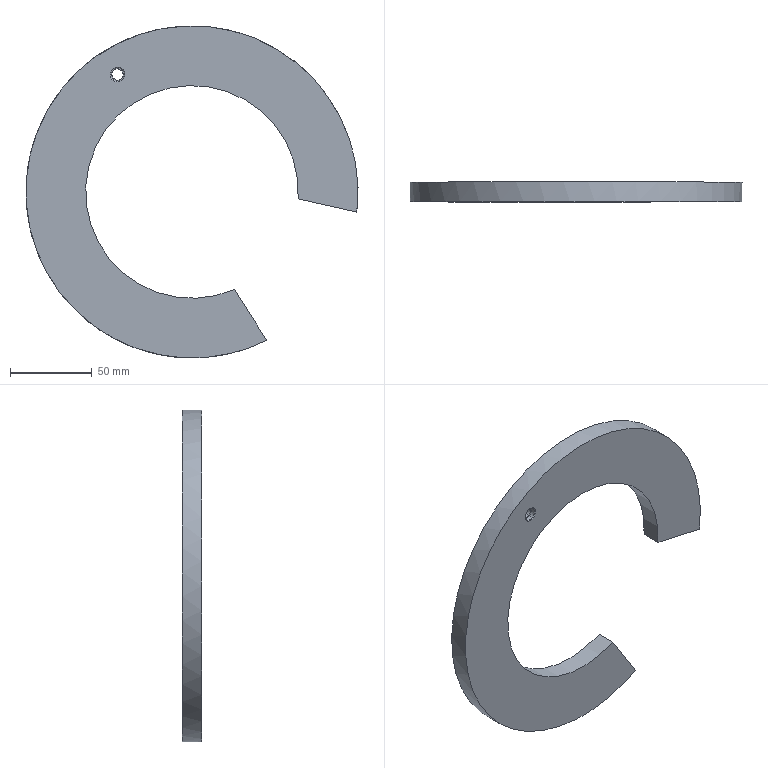Component | SolidWorks | Turntable-1 | 1 solid | 13 faces | box 203 x 12 x 203 mm | volume 191203 mm3 | cylinder 6 | plane 5 | cone 2 | commonest cylinder face diameters 8 x2 6.8 x2 130 x1 203 x1
STEP:
#1=CARTESIAN_POINT('',(1.076,-1.949,9.179));
#2=VERTEX_POINT('',#1);
#3=CARTESIAN_POINT('',(1.245,-1.949,8.913));
#4=VERTEX_POINT('',#3);
#5=CARTESIAN_POINT('',(1.16,-1.949,9.046));
#6=DIRECTION('',(0.,-1.,0.));
#7=DIRECTION('',(0.5356,0.,-0.8445));
#8=AXIS2_PLACEMENT_3D('',#5,#6,#7);
#9=CIRCLE('',#8,0.1575);
#10=EDGE_CURVE('',#2,#4,#9,.T.);
#11=ORIENTED_EDGE('',*,*,#10,.F.);
#12=CARTESIAN_POINT('',(1.076,-2.05,9.179));
#13=VERTEX_POINT('',#12);
#14=CARTESIAN_POINT('',(1.076,-1.949,9.179));
#15=DIRECTION('',(0.,-1.,0.));
#16=VECTOR('',#15,39.37);
#17=LINE('',#14,#16);
#18=EDGE_CURVE('',#2,#13,#17,.T.);
#19=ORIENTED_EDGE('',*,*,#18,.T.);
#20=CARTESIAN_POINT('',(1.245,-2.05,8.913));
#21=VERTEX_POINT('',#20);
#22=CARTESIAN_POINT('',(1.16,-2.05,9.046));
#23=DIRECTION('',(0.,1.,0.));
#24=DIRECTION('',(0.5356,0.,-0.8445));
#25=AXIS2_PLACEMENT_3D('',#22,#23,#24);
#26=CIRCLE('',#25,0.1575);
#27=EDGE_CURVE('',#21,#13,#26,.T.);
#28=ORIENTED_EDGE('',*,*,#27,.F.);
#29=CARTESIAN_POINT('',(1.245,-1.949,8.913));
#30=DIRECTION('',(0.,-1.,0.));
#31=VECTOR('',#30,39.37);
#32=LINE('',#29,#31);
#33=EDGE_CURVE('',#4,#21,#32,.T.);
#34=ORIENTED_EDGE('',*,*,#33,.F.);
#35=EDGE_LOOP('',(#11,#19,#28,#34));
#36=FACE_OUTER_BOUND('',#35,.T.);
#37=CARTESIAN_POINT('',(1.16,-1.949,9.046));
#38=DIRECTION('',(0.,-1.,0.));
#39=DIRECTION('',(0.5356,0.,-0.8445));
#40=AXIS2_PLACEMENT_3D('',#37,#38,#39);
#41=CYLINDRICAL_SURFACE('',#40,0.1575);
#42=ADVANCED_FACE('',(#36),#41,.F.);
#43=ORIENTED_EDGE('',*,*,#27,.T.);
#44=CARTESIAN_POINT('',(1.065,-2.067,9.197));
#45=VERTEX_POINT('',#44);
#46=CARTESIAN_POINT('',(1.065,-2.067,9.197));
#47=DIRECTION('',(-0.4103,-0.6428,0.6469));
#48=VECTOR('',#47,39.37);
#49=LINE('',#46,#48);
#50=EDGE_CURVE('',#13,#45,#49,.T.);
#51=ORIENTED_EDGE('',*,*,#50,.T.);
#52=CARTESIAN_POINT('',(1.256,-2.067,8.896));
#53=VERTEX_POINT('',#52);
#54=CARTESIAN_POINT('',(1.16,-2.067,9.046));
#55=DIRECTION('',(0.,-1.,0.));
#56=DIRECTION('',(0.5356,0.,-0.8445));
#57=AXIS2_PLACEMENT_3D('',#54,#55,#56);
#58=CIRCLE('',#57,0.1781);
#59=EDGE_CURVE('',#45,#53,#58,.T.);
#60=ORIENTED_EDGE('',*,*,#59,.T.);
#61=CARTESIAN_POINT('',(1.256,-2.067,8.896));
#62=DIRECTION('',(0.4103,-0.6428,-0.6469));
#63=VECTOR('',#62,39.37);
#64=LINE('',#61,#63);
#65=EDGE_CURVE('',#21,#53,#64,.T.);
#66=ORIENTED_EDGE('',*,*,#65,.F.);
#67=EDGE_LOOP('',(#43,#51,#60,#66));
#68=FACE_OUTER_BOUND('',#67,.T.);
#69=CARTESIAN_POINT('',(1.16,-2.067,9.046));
#70=DIRECTION('',(0.,-1.,0.));
#71=DIRECTION('',(0.5356,0.,-0.8445));
#72=AXIS2_PLACEMENT_3D('',#69,#70,#71);
#73=CONICAL_SURFACE('',#72,0.1781,0.8727);
#74=ADVANCED_FACE('',(#68),#73,.F.);
#75=CARTESIAN_POINT('',(1.089,-1.594,9.16));
#76=VERTEX_POINT('',#75);
#77=CARTESIAN_POINT('',(1.232,-1.594,8.933));
#78=VERTEX_POINT('',#77);
#79=CARTESIAN_POINT('',(1.16,-1.594,9.046));
#80=DIRECTION('',(0.,-1.,0.));
#81=DIRECTION('',(0.5356,0.,-0.8445));
#82=AXIS2_PLACEMENT_3D('',#79,#80,#81);
#83=CIRCLE('',#82,0.1339);
#84=EDGE_CURVE('',#76,#78,#83,.T.);
#85=ORIENTED_EDGE('',*,*,#84,.F.);
#86=CARTESIAN_POINT('',(1.089,-1.949,9.16));
#87=VERTEX_POINT('',#86);
#88=CARTESIAN_POINT('',(1.089,-2.067,9.16));
#89=DIRECTION('',(0.,-1.,0.));
#90=VECTOR('',#89,39.37);
#91=LINE('',#88,#90);
#92=EDGE_CURVE('',#76,#87,#91,.T.);
#93=ORIENTED_EDGE('',*,*,#92,.T.);
#94=CARTESIAN_POINT('',(1.232,-1.949,8.933));
#95=VERTEX_POINT('',#94);
#96=CARTESIAN_POINT('',(1.16,-1.949,9.046));
#97=DIRECTION('',(0.,1.,0.));
#98=DIRECTION('',(0.5356,0.,-0.8445));
#99=AXIS2_PLACEMENT_3D('',#96,#97,#98);
#100=CIRCLE('',#99,0.1339);
#101=EDGE_CURVE('',#95,#87,#100,.T.);
#102=ORIENTED_EDGE('',*,*,#101,.F.);
#103=CARTESIAN_POINT('',(1.232,-2.067,8.933));
#104=DIRECTION('',(0.,-1.,0.));
#105=VECTOR('',#104,39.37);
#106=LINE('',#103,#105);
#107=EDGE_CURVE('',#78,#95,#106,.T.);
#108=ORIENTED_EDGE('',*,*,#107,.F.);
#109=EDGE_LOOP('',(#85,#93,#102,#108));
#110=FACE_OUTER_BOUND('',#109,.T.);
#111=CARTESIAN_POINT('',(1.16,-2.067,9.046));
#112=DIRECTION('',(0.,-1.,0.));
#113=DIRECTION('',(0.5356,0.,-0.8445));
#114=AXIS2_PLACEMENT_3D('',#111,#112,#113);
#115=CYLINDRICAL_SURFACE('',#114,0.1339);
#116=ADVANCED_FACE('',(#110),#115,.F.);
#117=ORIENTED_EDGE('',*,*,#92,.F.);
#118=CARTESIAN_POINT('',(1.16,-1.594,9.046));
#119=DIRECTION('',(0.,-1.,0.));
#120=DIRECTION('',(0.5356,0.,-0.8445));
#121=AXIS2_PLACEMENT_3D('',#118,#119,#120);
#122=CIRCLE('',#121,0.1339);
#123=EDGE_CURVE('',#78,#76,#122,.T.);
#124=ORIENTED_EDGE('',*,*,#123,.F.);
#125=ORIENTED_EDGE('',*,*,#107,.T.);
#126=CARTESIAN_POINT('',(1.16,-1.949,9.046));
#127=DIRECTION('',(0.,1.,0.));
#128=DIRECTION('',(0.5356,0.,-0.8445));
#129=AXIS2_PLACEMENT_3D('',#126,#127,#128);
#130=CIRCLE('',#129,0.1339);
#131=EDGE_CURVE('',#87,#95,#130,.T.);
#132=ORIENTED_EDGE('',*,*,#131,.F.);
#133=EDGE_LOOP('',(#117,#124,#125,#132));
#134=FACE_OUTER_BOUND('',#133,.T.);
#135=CARTESIAN_POINT('',(1.16,-2.067,9.046));
#136=DIRECTION('',(0.,-1.,0.));
#137=DIRECTION('',(0.5356,0.,-0.8445));
#138=AXIS2_PLACEMENT_3D('',#135,#136,#137);
#139=CYLINDRICAL_SURFACE('',#138,0.1339);
#140=ADVANCED_FACE('',(#134),#139,.F.);
#141=CARTESIAN_POINT('',(1.16,-2.067,9.046));
#142=DIRECTION('',(0.,-1.,0.));
#143=DIRECTION('',(0.5356,0.,-0.8445));
#144=AXIS2_PLACEMENT_3D('',#141,#142,#143);
#145=CIRCLE('',#144,0.1781);
#146=EDGE_CURVE('',#53,#45,#145,.T.);
#147=ORIENTED_EDGE('',*,*,#146,.F.);
#148=ORIENTED_EDGE('',*,*,#59,.F.);
#149=EDGE_LOOP('',(#147,#148));
#150=FACE_BOUND('',#149,.T.);
#151=CARTESIAN_POINT('',(6.919,-2.067,5.736));
#152=VERTEX_POINT('',#151);
#153=CARTESIAN_POINT('',(5.506,-2.067,6.052));
#154=VERTEX_POINT('',#153);
#155=CARTESIAN_POINT('',(5.506,-2.067,6.052));
#156=DIRECTION('',(-0.9759,0.,0.2184));
#157=VECTOR('',#156,39.37);
#158=LINE('',#155,#157);
#159=EDGE_CURVE('',#152,#154,#158,.T.);
#160=ORIENTED_EDGE('',*,*,#159,.F.);
#161=CARTESIAN_POINT('',(4.75,-2.067,2.651));
#162=VERTEX_POINT('',#161);
#163=CARTESIAN_POINT('',(6.919,-2.067,5.736));
#164=CARTESIAN_POINT('',(6.933,-2.067,5.845));
#165=CARTESIAN_POINT('',(6.942,-2.067,5.955));
#166=CARTESIAN_POINT('',(6.948,-2.067,6.121));
#167=CARTESIAN_POINT('',(6.949,-2.067,6.176));
#168=CARTESIAN_POINT('',(6.949,-2.067,6.287));
#169=CARTESIAN_POINT('',(6.945,-2.067,6.452));
#170=CARTESIAN_POINT('',(6.931,-2.067,6.617));
#171=CARTESIAN_POINT('',(6.903,-2.067,6.836));
#172=CARTESIAN_POINT('',(6.884,-2.067,6.945));
#173=CARTESIAN_POINT('',(6.838,-2.067,7.161));
#174=CARTESIAN_POINT('',(6.797,-2.067,7.321));
#175=CARTESIAN_POINT('',(6.746,-2.067,7.478));
#176=CARTESIAN_POINT('',(6.71,-2.067,7.582));
#177=CARTESIAN_POINT('',(6.691,-2.067,7.634));
#178=CARTESIAN_POINT('',(6.589,-2.067,7.891));
#179=CARTESIAN_POINT('',(6.492,-2.067,8.089));
#180=CARTESIAN_POINT('',(6.35,-2.067,8.326));
#181=CARTESIAN_POINT('',(6.32,-2.067,8.373));
#182=CARTESIAN_POINT('',(6.259,-2.067,8.465));
#183=CARTESIAN_POINT('',(6.166,-2.067,8.601));
#184=CARTESIAN_POINT('',(6.03,-2.067,8.775));
#185=CARTESIAN_POINT('',(5.92,-2.067,8.898));
#186=CARTESIAN_POINT('',(5.844,-2.067,8.979));
#187=CARTESIAN_POINT('',(5.806,-2.067,9.019));
#188=CARTESIAN_POINT('',(5.688,-2.067,9.136));
#189=CARTESIAN_POINT('',(5.526,-2.067,9.284));
#190=CARTESIAN_POINT('',(5.351,-2.067,9.419));
#191=CARTESIAN_POINT('',(5.17,-2.067,9.547));
#192=CARTESIAN_POINT('',(5.077,-2.067,9.607));
#193=CARTESIAN_POINT('',(4.888,-2.067,9.719));
#194=CARTESIAN_POINT('',(4.791,-2.067,9.771));
#195=CARTESIAN_POINT('',(4.641,-2.067,9.843));
#196=CARTESIAN_POINT('',(4.591,-2.067,9.866));
#197=CARTESIAN_POINT('',(4.49,-2.067,9.91));
#198=CARTESIAN_POINT('',(4.336,-2.067,9.972));
#199=CARTESIAN_POINT('',(4.128,-2.067,10.043));
#200=CARTESIAN_POINT('',(3.968,-2.067,10.086));
#201=CARTESIAN_POINT('',(3.861,-2.067,10.112));
#202=CARTESIAN_POINT('',(3.807,-2.067,10.125));
#203=CARTESIAN_POINT('',(3.536,-2.067,10.18));
#204=CARTESIAN_POINT('',(3.317,-2.067,10.206));
#205=CARTESIAN_POINT('',(3.041,-2.067,10.216));
#206=CARTESIAN_POINT('',(2.986,-2.067,10.217));
#207=CARTESIAN_POINT('',(2.875,-2.067,10.216));
#208=CARTESIAN_POINT('',(2.71,-2.067,10.212));
#209=CARTESIAN_POINT('',(2.545,-2.067,10.197));
#210=CARTESIAN_POINT('',(2.327,-2.067,10.169));
#211=CARTESIAN_POINT('',(2.217,-2.067,10.15));
#212=CARTESIAN_POINT('',(2.002,-2.067,10.103));
#213=CARTESIAN_POINT('',(1.842,-2.067,10.062));
#214=CARTESIAN_POINT('',(1.685,-2.067,10.01));
#215=CARTESIAN_POINT('',(1.58,-2.067,9.974));
#216=CARTESIAN_POINT('',(1.529,-2.067,9.955));
#217=CARTESIAN_POINT('',(1.374,-2.067,9.893));
#218=CARTESIAN_POINT('',(1.173,-2.067,9.804));
#219=CARTESIAN_POINT('',(0.9799,-2.067,9.697));
#220=CARTESIAN_POINT('',(0.8381,-2.067,9.612));
#221=CARTESIAN_POINT('',(0.7913,-2.067,9.582));
#222=CARTESIAN_POINT('',(0.6992,-2.067,9.521));
#223=CARTESIAN_POINT('',(0.5632,-2.067,9.427));
#224=CARTESIAN_POINT('',(0.3902,-2.067,9.29));
#225=CARTESIAN_POINT('',(0.2669,-2.067,9.18));
#226=CARTESIAN_POINT('',(0.186,-2.067,9.104));
#227=CARTESIAN_POINT('',(0.1464,-2.067,9.066));
#228=CARTESIAN_POINT('',(-0.04746,-2.067,8.869));
#229=CARTESIAN_POINT('',(-0.1887,-2.067,8.7));
#230=CARTESIAN_POINT('',(-0.4433,-2.067,8.338));
#231=CARTESIAN_POINT('',(-0.5547,-2.067,8.148));
#232=CARTESIAN_POINT('',(-0.674,-2.067,7.899));
#233=CARTESIAN_POINT('',(-0.6969,-2.067,7.849));
#234=CARTESIAN_POINT('',(-0.7406,-2.067,7.747));
#235=CARTESIAN_POINT('',(-0.8028,-2.067,7.594));
#236=CARTESIAN_POINT('',(-0.8727,-2.067,7.385));
#237=CARTESIAN_POINT('',(-0.9154,-2.067,7.225));
#238=CARTESIAN_POINT('',(-0.9417,-2.067,7.118));
#239=CARTESIAN_POINT('',(-0.9537,-2.067,7.064));
#240=CARTESIAN_POINT('',(-0.9865,-2.067,6.901));
#241=CARTESIAN_POINT('',(-1.021,-2.067,6.683));
#242=CARTESIAN_POINT('',(-1.037,-2.067,6.464));
#243=CARTESIAN_POINT('',(-1.043,-2.067,6.298));
#244=CARTESIAN_POINT('',(-1.044,-2.067,6.242));
#245=CARTESIAN_POINT('',(-1.043,-2.067,6.132));
#246=CARTESIAN_POINT('',(-1.038,-2.067,5.967));
#247=CARTESIAN_POINT('',(-1.023,-2.067,5.802));
#248=CARTESIAN_POINT('',(-0.9938,-2.067,5.583));
#249=CARTESIAN_POINT('',(-0.9746,-2.067,5.474));
#250=CARTESIAN_POINT('',(-0.9275,-2.067,5.259));
#251=CARTESIAN_POINT('',(-0.8855,-2.067,5.099));
#252=CARTESIAN_POINT('',(-0.8337,-2.067,4.942));
#253=CARTESIAN_POINT('',(-0.7969,-2.067,4.838));
#254=CARTESIAN_POINT('',(-0.7774,-2.067,4.786));
#255=CARTESIAN_POINT('',(-0.6746,-2.067,4.529));
#256=CARTESIAN_POINT('',(-0.5761,-2.067,4.332));
#257=CARTESIAN_POINT('',(-0.4325,-2.067,4.096));
#258=CARTESIAN_POINT('',(-0.4027,-2.067,4.05));
#259=CARTESIAN_POINT('',(-0.3415,-2.067,3.958));
#260=CARTESIAN_POINT('',(-0.2469,-2.067,3.822));
#261=CARTESIAN_POINT('',(-0.1099,-2.067,3.649));
#262=CARTESIAN_POINT('',(0.0008713,-2.067,3.526));
#263=CARTESIAN_POINT('',(0.07655,-2.067,3.446));
#264=CARTESIAN_POINT('',(0.1152,-2.067,3.406));
#265=CARTESIAN_POINT('',(0.2334,-2.067,3.29));
#266=CARTESIAN_POINT('',(0.3152,-2.067,3.216));
#267=CARTESIAN_POINT('',(0.4847,-2.067,3.076));
#268=CARTESIAN_POINT('',(0.5725,-2.067,3.009));
#269=CARTESIAN_POINT('',(0.7538,-2.067,2.882));
#270=CARTESIAN_POINT('',(0.9397,-2.067,2.763));
#271=CARTESIAN_POINT('',(1.135,-2.067,2.66));
#272=CARTESIAN_POINT('',(1.284,-2.067,2.589));
#273=CARTESIAN_POINT('',(1.335,-2.067,2.566));
#274=CARTESIAN_POINT('',(1.436,-2.067,2.523));
#275=CARTESIAN_POINT('',(1.59,-2.067,2.461));
#276=CARTESIAN_POINT('',(1.799,-2.067,2.392));
#277=CARTESIAN_POINT('',(1.959,-2.067,2.35));
#278=CARTESIAN_POINT('',(2.066,-2.067,2.324));
#279=CARTESIAN_POINT('',(2.12,-2.067,2.312));
#280=CARTESIAN_POINT('',(2.391,-2.067,2.258));
#281=CARTESIAN_POINT('',(2.61,-2.067,2.233));
#282=CARTESIAN_POINT('',(2.887,-2.067,2.225));
#283=CARTESIAN_POINT('',(2.942,-2.067,2.224));
#284=CARTESIAN_POINT('',(3.052,-2.067,2.225));
#285=CARTESIAN_POINT('',(3.217,-2.067,2.23));
#286=CARTESIAN_POINT('',(3.382,-2.067,2.246));
#287=CARTESIAN_POINT('',(3.546,-2.067,2.268));
#288=CARTESIAN_POINT('',(3.601,-2.067,2.277));
#289=CARTESIAN_POINT('',(3.71,-2.067,2.296));
#290=CARTESIAN_POINT('',(3.872,-2.067,2.329));
#291=CARTESIAN_POINT('',(4.085,-2.067,2.385));
#292=CARTESIAN_POINT('',(4.242,-2.067,2.438));
#293=CARTESIAN_POINT('',(4.346,-2.067,2.475));
#294=CARTESIAN_POINT('',(4.398,-2.067,2.494));
#295=CARTESIAN_POINT('',(4.551,-2.067,2.556));
#296=CARTESIAN_POINT('',(4.652,-2.067,2.602));
#297=CARTESIAN_POINT('',(4.75,-2.067,2.651));
#298=B_SPLINE_CURVE_WITH_KNOTS('',3,(#163,#164,#165,#166,#167,#168,#169,#170,#171,#172,#173,#174,#175,#176,#177,#178,#179,#180,#181,#182,#183,#184,#185,#186,#187,#188,#189,#190,#191,#192,#193,#194,#195,#196,#197,#198,#199,#200,#201,#202,#203,#204,#205,#206,#207,#208,#209,#210,#211,#212,#213,#214,#215,#216,#217,#218,#219,#220,#221,#222,#223,#224,#225,#226,#227,#228,#229,#230,#231,#232,#233,#234,#235,#236,#237,#238,#239,#240,#241,#242,#243,#244,#245,#246,#247,#248,#249,#250,#251,#252,#253,#254,#255,#256,#257,#258,#259,#260,#261,#262,#263,#264,#265,#266,#267,#268,#269,#270,#271,#272,#273,#274,#275,#276,#277,#278,#279,#280,#281,#282,#283,#284,#285,#286,#287,#288,#289,#290,#291,#292,#293,#294,#295,#296,#297),.UNSPECIFIED.,.F.,.F.,(4,2,2,1,2,2,1,2,2,2,2,1,1,2,2,1,2,2,2,2,1,1,2,2,2,2,1,2,2,1,2,2,1,2,2,1,1,2,2,2,2,2,1,1,2,2,1,2,2,1,2,2,1,2,2,2,2,1,1,2,2,2,2,1,2,2,1,1,2,2,2,2,1,2,2,1,1,2,2,4),(0.1407,0.1539,0.1605,0.1671,0.1802,0.1934,0.2066,0.2132,0.2198,0.2462,0.2527,0.2593,0.2725,0.2791,0.2857,0.2989,0.3121,0.3252,0.3384,0.345,0.3516,0.3648,0.3714,0.378,0.4043,0.4109,0.4175,0.4307,0.4439,0.4571,0.4636,0.4702,0.4834,0.4966,0.5032,0.5098,0.523,0.5295,0.5361,0.5625,0.5889,0.5955,0.602,0.6152,0.6218,0.6284,0.6416,0.6548,0.6614,0.6679,0.6811,0.6943,0.7075,0.7141,0.7207,0.747,0.7536,0.7602,0.7734,0.78,0.7866,0.7998,0.8129,0.8261,0.8393,0.8459,0.8525,0.8657,0.8723,0.8788,0.9052,0.9118,0.9184,0.9316,0.9382,0.9448,0.9579,0.9645,0.9711,0.9843),.UNSPECIFIED.);
#299=EDGE_CURVE('',#152,#162,#298,.T.);
#300=ORIENTED_EDGE('',*,*,#299,.T.);
#301=CARTESIAN_POINT('',(3.975,-2.067,3.874));
#302=VERTEX_POINT('',#301);
#303=CARTESIAN_POINT('',(3.975,-2.067,3.874));
#304=DIRECTION('',(0.5356,0.,-0.8445));
#305=VECTOR('',#304,39.37);
#306=LINE('',#303,#305);
#307=EDGE_CURVE('',#302,#162,#306,.T.);
#308=ORIENTED_EDGE('',*,*,#307,.F.);
#309=CARTESIAN_POINT('',(2.953,-2.067,6.22));
#310=DIRECTION('',(0.,-1.,0.));
#311=DIRECTION('',(0.5356,0.,-0.8445));
#312=AXIS2_PLACEMENT_3D('',#309,#310,#311);
#313=CIRCLE('',#312,2.559);
#314=EDGE_CURVE('',#154,#302,#313,.T.);
#315=ORIENTED_EDGE('',*,*,#314,.F.);
#316=EDGE_LOOP('',(#160,#300,#308,#315));
#317=FACE_OUTER_BOUND('',#316,.T.);
#318=CARTESIAN_POINT('',(2.953,-2.067,6.22));
#319=DIRECTION('',(0.,-1.,0.));
#320=DIRECTION('',(0.5356,0.,-0.8445));
#321=AXIS2_PLACEMENT_3D('',#318,#319,#320);
#322=PLANE('',#321);
#323=ADVANCED_FACE('',(#150,#317),#322,.T.);
#324=CARTESIAN_POINT('',(4.75,-1.594,2.651));
#325=VERTEX_POINT('',#324);
#326=CARTESIAN_POINT('',(4.75,-1.594,2.651));
#327=DIRECTION('',(0.,-1.,0.));
#328=VECTOR('',#327,39.37);
#329=LINE('',#326,#328);
#330=EDGE_CURVE('',#325,#162,#329,.T.);
#331=ORIENTED_EDGE('',*,*,#330,.F.);
#332=CARTESIAN_POINT('',(3.975,-1.594,3.874));
#333=VERTEX_POINT('',#332);
#334=CARTESIAN_POINT('',(3.975,-1.594,3.874));
#335=DIRECTION('',(0.5356,0.,-0.8445));
#336=VECTOR('',#335,39.37);
#337=LINE('',#334,#336);
#338=EDGE_CURVE('',#333,#325,#337,.T.);
#339=ORIENTED_EDGE('',*,*,#338,.F.);
#340=CARTESIAN_POINT('',(3.975,-1.594,3.874));
#341=DIRECTION('',(0.,-1.,0.));
#342=VECTOR('',#341,39.37);
#343=LINE('',#340,#342);
#344=EDGE_CURVE('',#333,#302,#343,.T.);
#345=ORIENTED_EDGE('',*,*,#344,.T.);
#346=ORIENTED_EDGE('',*,*,#307,.T.);
#347=EDGE_LOOP('',(#331,#339,#345,#346));
#348=FACE_OUTER_BOUND('',#347,.T.);
#349=CARTESIAN_POINT('',(3.975,-1.594,3.874));
#350=DIRECTION('',(-0.8445,0.,-0.5356));
#351=DIRECTION('',(0.,1.,0.));
#352=AXIS2_PLACEMENT_3D('',#349,#350,#351);
#353=PLANE('',#352);
#354=ADVANCED_FACE('',(#348),#353,.F.);
#355=CARTESIAN_POINT('',(6.919,-1.594,5.736));
#356=VERTEX_POINT('',#355);
#357=CARTESIAN_POINT('',(6.919,-1.594,5.736));
#358=DIRECTION('',(0.,1.,0.));
#359=VECTOR('',#358,39.37);
#360=LINE('',#357,#359);
#361=EDGE_CURVE('',#152,#356,#360,.T.);
#362=ORIENTED_EDGE('',*,*,#361,.F.);
#363=ORIENTED_EDGE('',*,*,#159,.T.);
#364=CARTESIAN_POINT('',(5.506,-1.594,6.052));
#365=VERTEX_POINT('',#364);
#366=CARTESIAN_POINT('',(5.506,-1.594,6.052));
#367=DIRECTION('',(0.,-1.,0.));
#368=VECTOR('',#367,39.37);
#369=LINE('',#366,#368);
#370=EDGE_CURVE('',#365,#154,#369,.T.);
#371=ORIENTED_EDGE('',*,*,#370,.F.);
#372=CARTESIAN_POINT('',(5.506,-1.594,6.052));
#373=DIRECTION('',(-0.9759,0.,0.2184));
#374=VECTOR('',#373,39.37);
#375=LINE('',#372,#374);
#376=EDGE_CURVE('',#356,#365,#375,.T.);
#377=ORIENTED_EDGE('',*,*,#376,.F.);
#378=EDGE_LOOP('',(#362,#363,#371,#377));
#379=FACE_OUTER_BOUND('',#378,.T.);
#380=CARTESIAN_POINT('',(5.506,-1.594,6.052));
#381=DIRECTION('',(0.2184,0.,0.9759));
#382=DIRECTION('',(0.,-1.,0.));
#383=AXIS2_PLACEMENT_3D('',#380,#381,#382);
#384=PLANE('',#383);
#385=ADVANCED_FACE('',(#379),#384,.F.);
#386=ORIENTED_EDGE('',*,*,#123,.T.);
#387=ORIENTED_EDGE('',*,*,#84,.T.);
#388=EDGE_LOOP('',(#386,#387));
#389=FACE_BOUND('',#388,.T.);
#390=CARTESIAN_POINT('',(2.953,-1.594,6.22));
#391=DIRECTION('',(0.,-1.,0.));
#392=DIRECTION('',(0.5356,0.,-0.8445));
#393=AXIS2_PLACEMENT_3D('',#390,#391,#392);
#394=CIRCLE('',#393,3.996);
#395=EDGE_CURVE('',#356,#325,#394,.T.);
#396=ORIENTED_EDGE('',*,*,#395,.F.);
#397=ORIENTED_EDGE('',*,*,#376,.T.);
#398=CARTESIAN_POINT('',(2.953,-1.594,6.22));
#399=DIRECTION('',(0.,-1.,0.));
#400=DIRECTION('',(0.5356,0.,-0.8445));
#401=AXIS2_PLACEMENT_3D('',#398,#399,#400);
#402=CIRCLE('',#401,2.559);
#403=EDGE_CURVE('',#365,#333,#402,.T.);
#404=ORIENTED_EDGE('',*,*,#403,.T.);
#405=ORIENTED_EDGE('',*,*,#338,.T.);
#406=EDGE_LOOP('',(#396,#397,#404,#405));
#407=FACE_OUTER_BOUND('',#406,.T.);
#408=CARTESIAN_POINT('',(2.953,-1.594,6.22));
#409=DIRECTION('',(0.,-1.,0.));
#410=DIRECTION('',(0.5356,0.,-0.8445));
#411=AXIS2_PLACEMENT_3D('',#408,#409,#410);
#412=PLANE('',#411);
#413=ADVANCED_FACE('',(#389,#407),#412,.F.);
#414=ORIENTED_EDGE('',*,*,#314,.T.);
#415=ORIENTED_EDGE('',*,*,#344,.F.);
#416=ORIENTED_EDGE('',*,*,#403,.F.);
#417=ORIENTED_EDGE('',*,*,#370,.T.);
#418=EDGE_LOOP('',(#414,#415,#416,#417));
#419=FACE_OUTER_BOUND('',#418,.T.);
#420=CARTESIAN_POINT('',(2.953,-1.594,6.22));
#421=DIRECTION('',(0.,-1.,0.));
#422=DIRECTION('',(0.5356,0.,-0.8445));
#423=AXIS2_PLACEMENT_3D('',#420,#421,#422);
#424=CYLINDRICAL_SURFACE('',#423,2.559);
#425=ADVANCED_FACE('',(#419),#424,.F.);
#426=ORIENTED_EDGE('',*,*,#50,.F.);
#427=CARTESIAN_POINT('',(1.16,-2.05,9.046));
#428=DIRECTION('',(0.,1.,0.));
#429=DIRECTION('',(0.5356,0.,-0.8445));
#430=AXIS2_PLACEMENT_3D('',#427,#428,#429);
#431=CIRCLE('',#430,0.1575);
#432=EDGE_CURVE('',#13,#21,#431,.T.);
#433=ORIENTED_EDGE('',*,*,#432,.T.);
#434=ORIENTED_EDGE('',*,*,#65,.T.);
#435=ORIENTED_EDGE('',*,*,#146,.T.);
#436=EDGE_LOOP('',(#426,#433,#434,#435));
#437=FACE_OUTER_BOUND('',#436,.T.);
#438=CARTESIAN_POINT('',(1.16,-2.067,9.046));
#439=DIRECTION('',(0.,-1.,0.));
#440=DIRECTION('',(0.5356,0.,-0.8445));
#441=AXIS2_PLACEMENT_3D('',#438,#439,#440);
#442=CONICAL_SURFACE('',#441,0.1781,0.8727);
#443=ADVANCED_FACE('',(#437),#442,.F.);
#444=ORIENTED_EDGE('',*,*,#330,.T.);
#445=ORIENTED_EDGE('',*,*,#299,.F.);
#446=ORIENTED_EDGE('',*,*,#361,.T.);
#447=ORIENTED_EDGE('',*,*,#395,.T.);
#448=EDGE_LOOP('',(#444,#445,#446,#447));
#449=FACE_OUTER_BOUND('',#448,.T.);
#450=CARTESIAN_POINT('',(2.953,-1.594,6.22));
#451=DIRECTION('',(0.,-1.,0.));
#452=DIRECTION('',(0.5356,0.,-0.8445));
#453=AXIS2_PLACEMENT_3D('',#450,#451,#452);
#454=CYLINDRICAL_SURFACE('',#453,3.996);
#455=ADVANCED_FACE('',(#449),#454,.T.);
#456=CARTESIAN_POINT('',(1.16,-1.949,9.046));
#457=DIRECTION('',(0.,-1.,0.));
#458=DIRECTION('',(0.5356,0.,-0.8445));
#459=AXIS2_PLACEMENT_3D('',#456,#457,#458);
#460=CIRCLE('',#459,0.1575);
#461=EDGE_CURVE('',#4,#2,#460,.T.);
#462=ORIENTED_EDGE('',*,*,#461,.T.);
#463=ORIENTED_EDGE('',*,*,#10,.T.);
#464=EDGE_LOOP('',(#462,#463));
#465=FACE_OUTER_BOUND('',#464,.T.);
#466=ORIENTED_EDGE('',*,*,#101,.T.);
#467=ORIENTED_EDGE('',*,*,#131,.T.);
#468=EDGE_LOOP('',(#466,#467));
#469=FACE_BOUND('',#468,.T.);
#470=CARTESIAN_POINT('',(1.16,-1.949,9.046));
#471=DIRECTION('',(0.,-1.,0.));
#472=DIRECTION('',(0.5356,0.,-0.8445));
#473=AXIS2_PLACEMENT_3D('',#470,#471,#472);
#474=PLANE('',#473);
#475=ADVANCED_FACE('',(#465,#469),#474,.T.);
#476=ORIENTED_EDGE('',*,*,#18,.F.);
#477=ORIENTED_EDGE('',*,*,#461,.F.);
#478=ORIENTED_EDGE('',*,*,#33,.T.);
#479=ORIENTED_EDGE('',*,*,#432,.F.);
#480=EDGE_LOOP('',(#476,#477,#478,#479));
#481=FACE_OUTER_BOUND('',#480,.T.);
#482=CARTESIAN_POINT('',(1.16,-1.949,9.046));
#483=DIRECTION('',(0.,-1.,0.));
#484=DIRECTION('',(0.5356,0.,-0.8445));
#485=AXIS2_PLACEMENT_3D('',#482,#483,#484);
#486=CYLINDRICAL_SURFACE('',#485,0.1575);
#487=ADVANCED_FACE('',(#481),#486,.F.);
#488=CLOSED_SHELL('',(#42,#74,#116,#140,#323,#354,#385,#413,#425,#443,#455,#475,#487));
#489=MANIFOLD_SOLID_BREP('',#488);
#490=CARTESIAN_POINT('',(0.,0.,0.));
#491=DIRECTION('',(0.,0.,1.));
#492=DIRECTION('',(1.,0.,0.));
#493=AXIS2_PLACEMENT_3D('',#490,#491,#492);
#494=(LENGTH_UNIT()NAMED_UNIT(*)SI_UNIT($,.METRE.));
#495=LENGTH_MEASURE_WITH_UNIT(LENGTH_MEASURE(0.0254),#494);
#496=DIMENSIONAL_EXPONENTS(1.,0.,0.,0.,0.,0.,0.);
#497=(CONVERSION_BASED_UNIT('',#495)LENGTH_UNIT()NAMED_UNIT(#496));
#498=UNCERTAINTY_MEASURE_WITH_UNIT(LENGTH_MEASURE(0.00001),#497,'','');
#499=(NAMED_UNIT(*)PLANE_ANGLE_UNIT()SI_UNIT($,.RADIAN.));
#500=(NAMED_UNIT(*)SI_UNIT($,.STERADIAN.)SOLID_ANGLE_UNIT());
#501=(GEOMETRIC_REPRESENTATION_CONTEXT(3)GLOBAL_UNCERTAINTY_ASSIGNED_CONTEXT((#498))GLOBAL_UNIT_ASSIGNED_CONTEXT((#497,#499,#500))REPRESENTATION_CONTEXT('',''));
#502=ADVANCED_BREP_SHAPE_REPRESENTATION('',(#489,#493),#501);
#503=COLOUR_RGB('',0.7922,0.8196,0.9333);
#504=FILL_AREA_STYLE_COLOUR('',#503);
#505=FILL_AREA_STYLE('',(#504));
#506=SURFACE_STYLE_FILL_AREA(#505);
#507=SURFACE_SIDE_STYLE('',(#506));
#508=SURFACE_STYLE_USAGE(.BOTH.,#507);
#509=PRESENTATION_STYLE_ASSIGNMENT((#508));
#510=STYLED_ITEM('',(#509),#489);
#511=(LENGTH_UNIT()NAMED_UNIT(*)SI_UNIT($,.METRE.));
#512=LENGTH_MEASURE_WITH_UNIT(LENGTH_MEASURE(0.0254),#511);
#513=DIMENSIONAL_EXPONENTS(1.,0.,0.,0.,0.,0.,0.);
#514=(CONVERSION_BASED_UNIT('',#512)LENGTH_UNIT()NAMED_UNIT(#513));
#515=UNCERTAINTY_MEASURE_WITH_UNIT(LENGTH_MEASURE(0.00001),#514,'','');
#516=(NAMED_UNIT(*)PLANE_ANGLE_UNIT()SI_UNIT($,.RADIAN.));
#517=(NAMED_UNIT(*)SI_UNIT($,.STERADIAN.)SOLID_ANGLE_UNIT());
#518=(GEOMETRIC_REPRESENTATION_CONTEXT(3)GLOBAL_UNCERTAINTY_ASSIGNED_CONTEXT((#515))GLOBAL_UNIT_ASSIGNED_CONTEXT((#514,#516,#517))REPRESENTATION_CONTEXT('',''));
#519=MECHANICAL_DESIGN_GEOMETRIC_PRESENTATION_REPRESENTATION('',(#510),#518);
#520=PRESENTATION_LAYER_ASSIGNMENT('','',(#510));